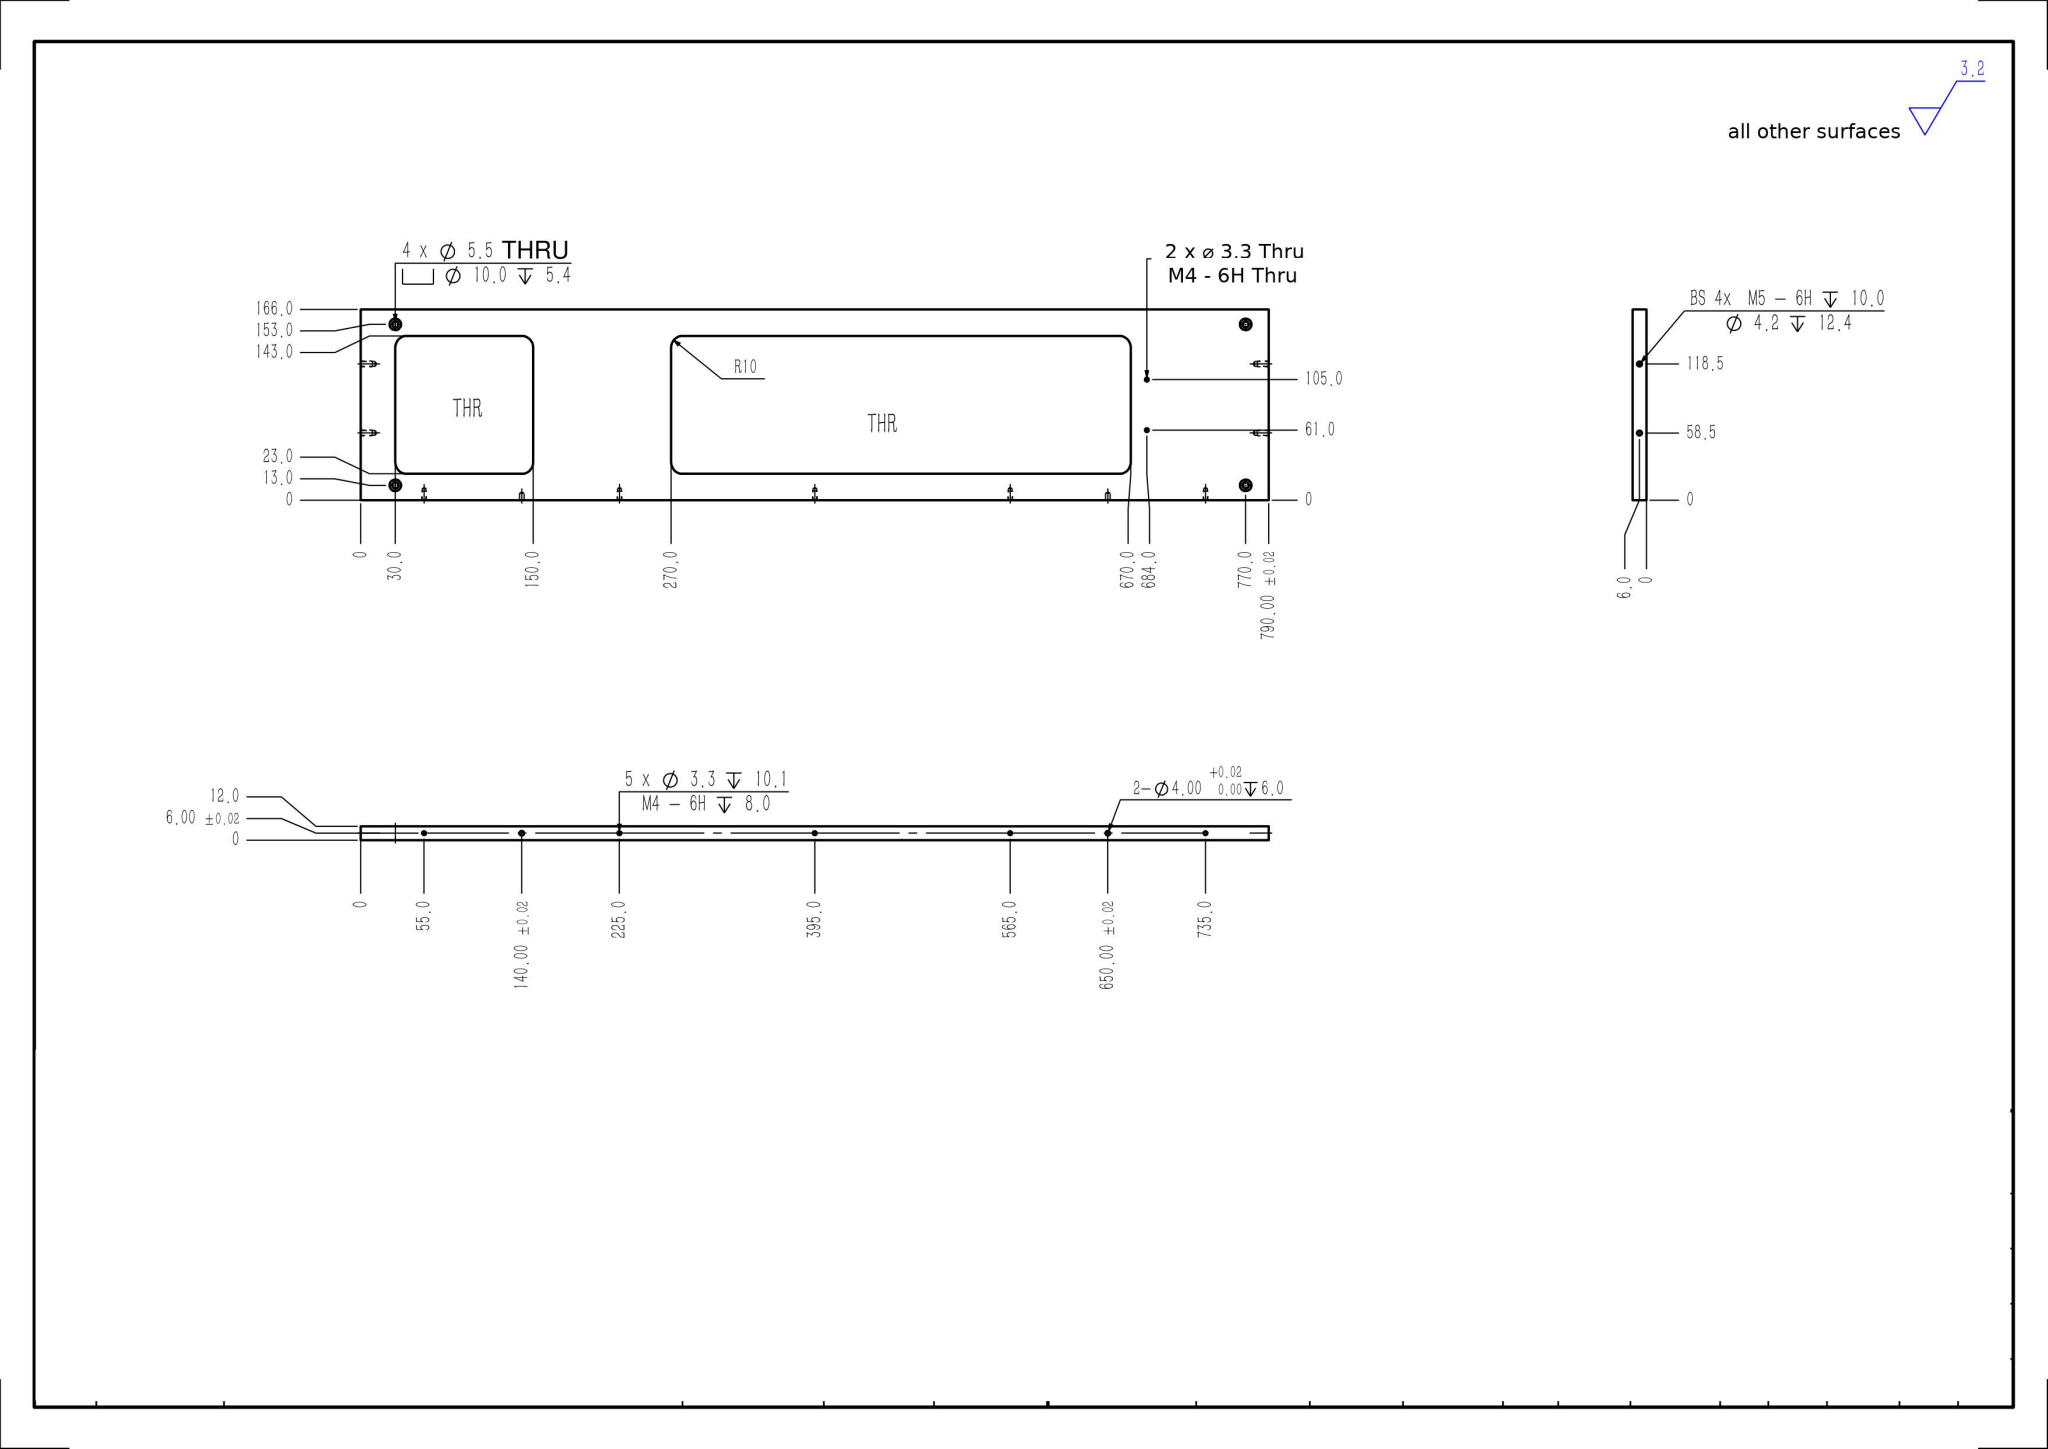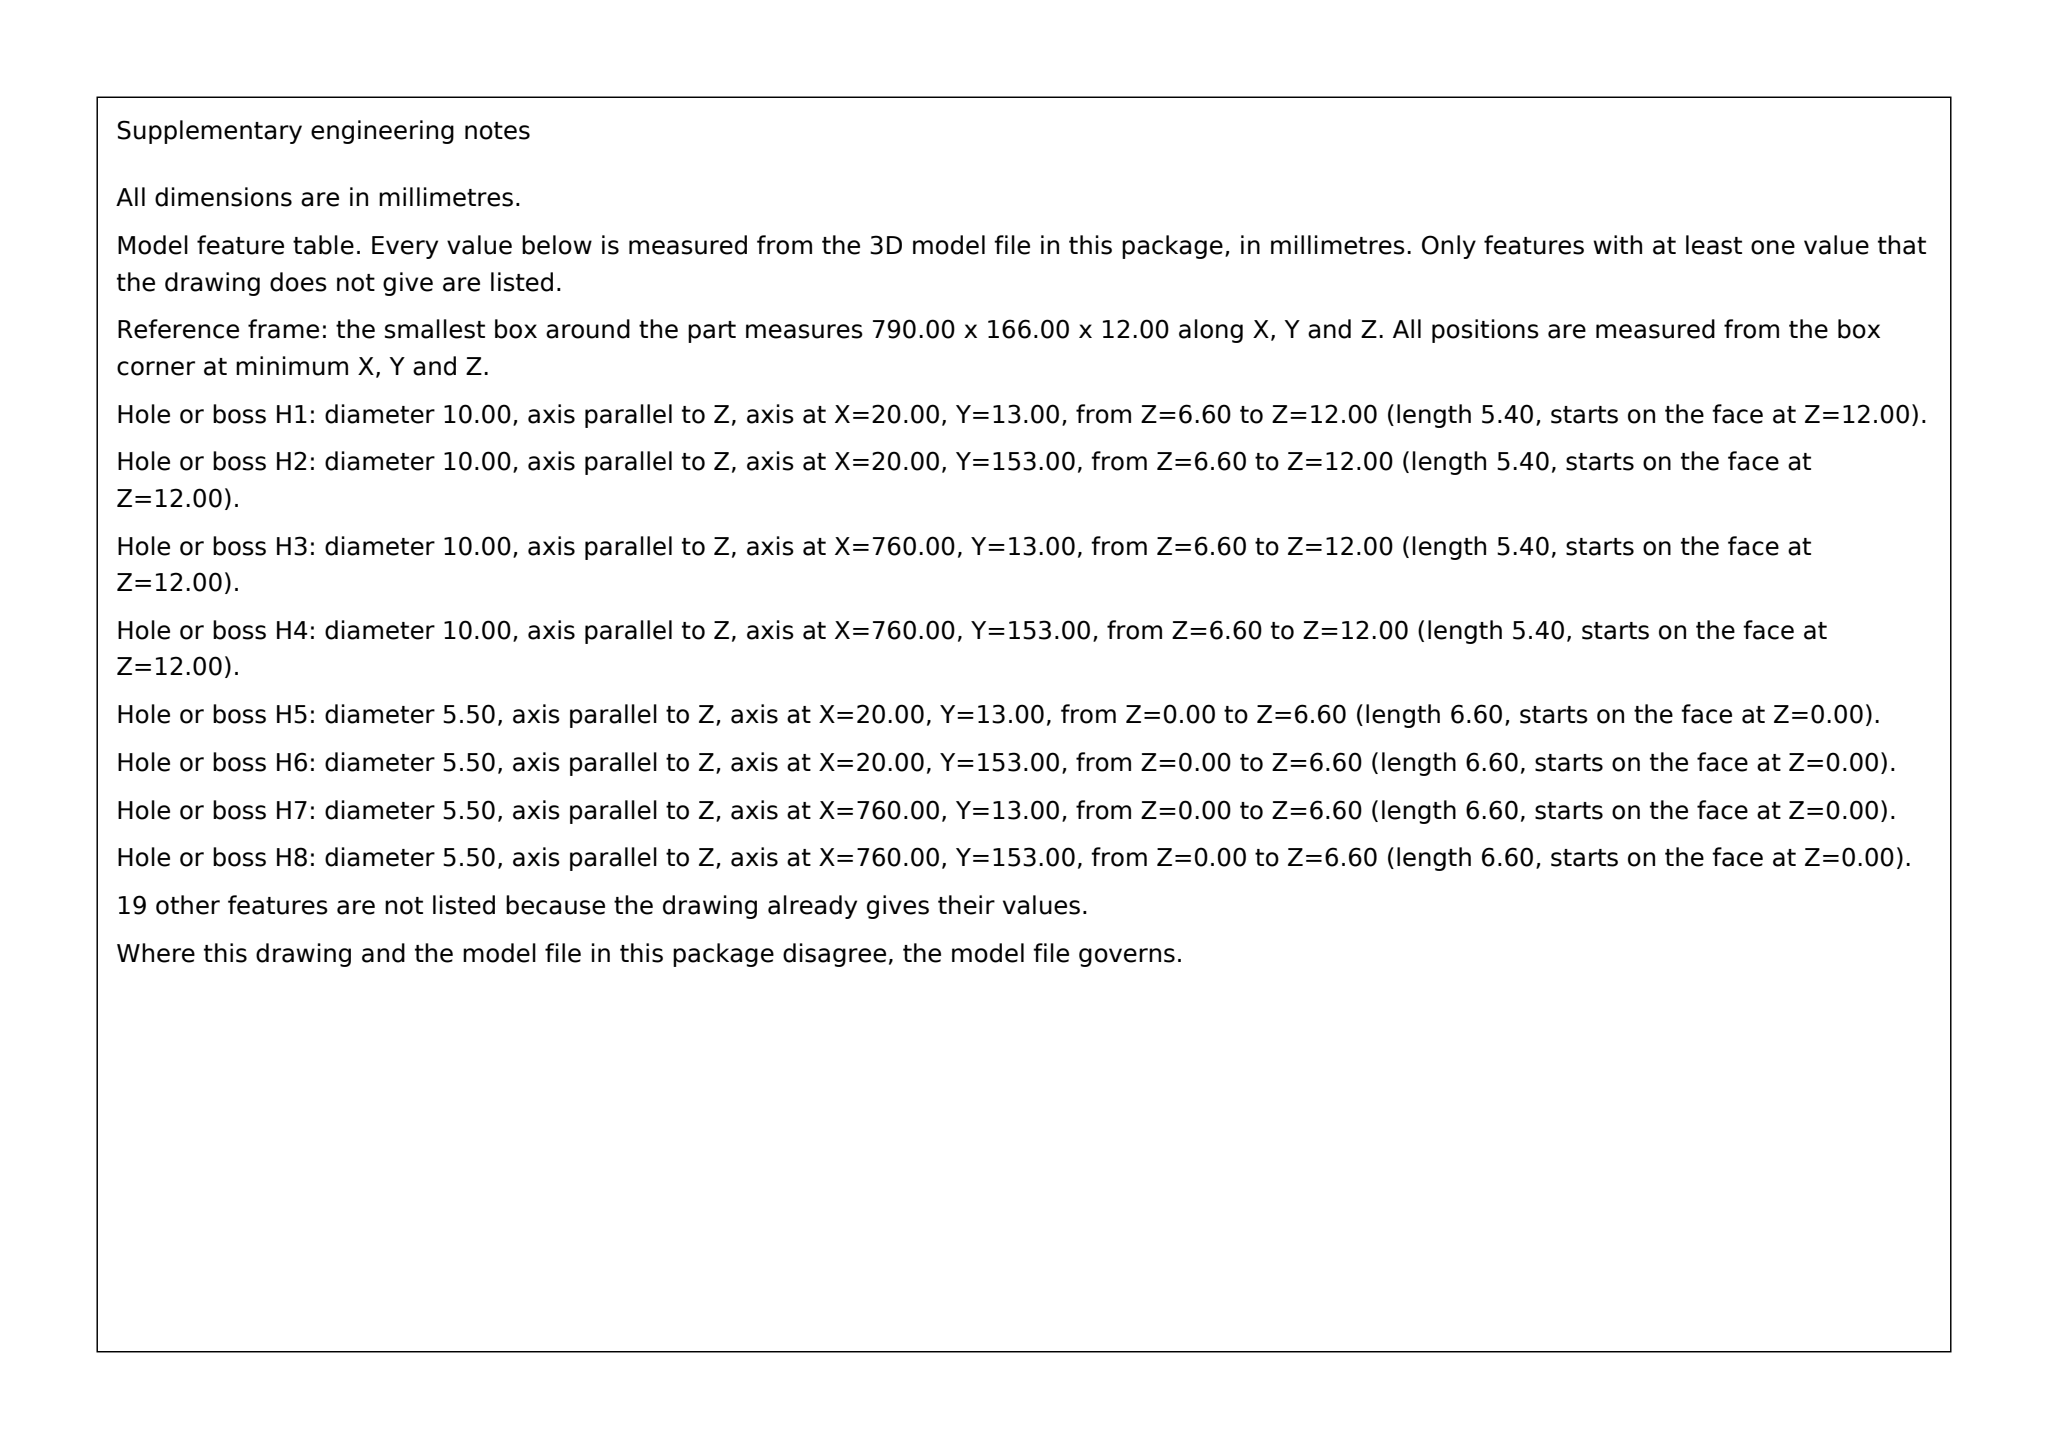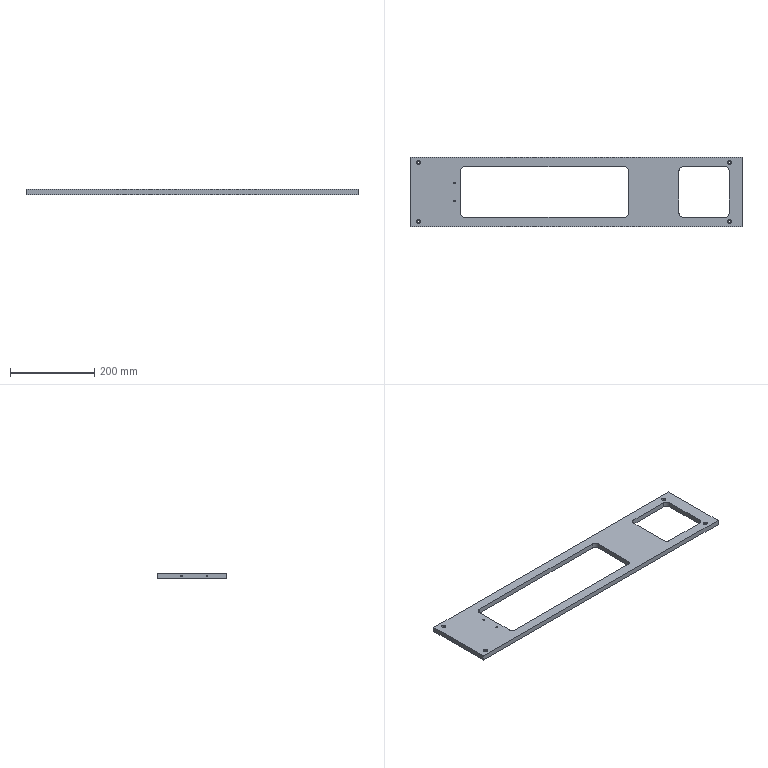Part | SolidWorks | mm | 1 solid | 90 faces | box 790 x 166 x 12 mm | volume 823094 mm3 | cylinder 50 | cone 22 | plane 18 | commonest cylinder face diameters 3.3 x14 4.2 x8 10 x8 5.5 x8 20 x8 4 x4
build123d program:
from build123d import *

# Parameters (mm, degrees)
SKETCH1_W                                       = 790
SKETCH1_H                                       = 166
BOSS_EXTRUDE1_DEPTH                             = 6
SKETCH63_W                                      = 120
SKETCH63_H                                      = 120
SKETCH63_W_2                                    = 400
CUT_EXTRUDE16_DEPTH                             = 404.804
FILLET6_R                                       = 10
M5_HEX_SOCKET_HEAD_CAP_SCREW_CBORE1_D           = 5.5
M5_HEX_SOCKET_HEAD_CAP_SCREW_CBORE1_CBORE_D     = 10
M5_HEX_SOCKET_HEAD_CAP_SCREW_CBORE1_CBORE_DEPTH = 5.4
M5_TAPPED_HOLE1_D                               = 4.2
M5_TAPPED_HOLE1_DEPTH                           = 12.4
M5_TAPPED_HOLE1_TIP                             = 1.262
M5_TAPPED_HOLE2_D                               = 4.2
M5_TAPPED_HOLE2_DEPTH                           = 12.4
M5_TAPPED_HOLE2_TIP                             = 1.262
M4_TAPPED_HOLE1_D                               = 3.3
M4_TAPPED_HOLE2_D                               = 3.3
M4_TAPPED_HOLE2_DEPTH                           = 10.1
M4_TAPPED_HOLE2_TIP                             = 0.9914
SIZE_MM_DOWEL_PIN_HOLE1_D                       = 4
SIZE_MM_DOWEL_PIN_HOLE1_DEPTH                   = 6
SIZE_MM_DOWEL_PIN_HOLE1_TIP                     = 1.202


with BuildPart() as part:
    # Sketch1 → Boss-Extrude1 (new, symmetric)
    with BuildSketch(Plane.XY):
        Rectangle(SKETCH1_W, SKETCH1_H)
    extrude(amount=BOSS_EXTRUDE1_DEPTH, both=True)

    # Sketch63 → Cut-Extrude16 (cut, through all)
    with BuildSketch(Plane(origin=(0, 0, -6), x_dir=(-1, 0, 0), z_dir=(0, 0, -1))):
        with Locations((-305, 0)):
            Rectangle(SKETCH63_W, SKETCH63_H)
        with Locations((75, 0)):
            Rectangle(SKETCH63_W_2, SKETCH63_H)
    extrude(amount=-CUT_EXTRUDE16_DEPTH, mode=Mode.SUBTRACT)

    # Fillet6
    fillet6_edges = [part.edges().sort_by_distance(p)[0] for p in [
        (245, 60, 0),
        (245, -60, 0),
        (365, -60, 0),
        (365, 60, 0),
        (-275, 60, 0),
        (-275, -60, 0),
        (125, -60, 0),
        (125, 60, 0),
    ]]
    fillet(fillet6_edges, radius=FILLET6_R)

    # M5 Hex Socket Head Cap Screw CBORE1 (through all)
    with Locations(Plane(origin=(0, 0, 6), x_dir=(-1, 0, 0), z_dir=(0, 0, 1))):
        with Locations((-365, -70), (-365, 70), (375, 70), (375, -70)):
            CounterBoreHole(M5_HEX_SOCKET_HEAD_CAP_SCREW_CBORE1_D / 2, M5_HEX_SOCKET_HEAD_CAP_SCREW_CBORE1_CBORE_D / 2, M5_HEX_SOCKET_HEAD_CAP_SCREW_CBORE1_CBORE_DEPTH)

    # M5 Tapped Hole1
    with Locations(Plane.ZY.offset(395)):
        with Locations((0, -35.5), (0, 24.5)):
            Hole(M5_TAPPED_HOLE1_D / 2, depth=M5_TAPPED_HOLE1_DEPTH)
            with Locations((0, 0, -(M5_TAPPED_HOLE1_DEPTH + M5_TAPPED_HOLE1_TIP / 2))):  # 118° drill point
                Cone(0, M5_TAPPED_HOLE1_D / 2, M5_TAPPED_HOLE1_TIP, mode=Mode.SUBTRACT)

    # M5 Tapped Hole2
    with Locations(Plane(origin=(395, 0, 0), x_dir=(0, 0, -1), z_dir=(1, 0, 0))):
        with Locations((0, 24.5), (0, -35.5)):
            Hole(M5_TAPPED_HOLE2_D / 2, depth=M5_TAPPED_HOLE2_DEPTH)
            with Locations((0, 0, -(M5_TAPPED_HOLE2_DEPTH + M5_TAPPED_HOLE2_TIP / 2))):  # 118° drill point
                Cone(0, M5_TAPPED_HOLE2_D / 2, M5_TAPPED_HOLE2_TIP, mode=Mode.SUBTRACT)

    # M4 Tapped Hole1 (through all)
    with Locations(Plane(origin=(0, 0, -6), x_dir=(-1, 0, 0), z_dir=(0, 0, -1))):
        with Locations((289, 22), (289, -22)):
            Hole(M4_TAPPED_HOLE1_D / 2)

    # M4 Tapped Hole2
    with Locations(Plane(origin=(0, 83, 0), x_dir=(1, 0, 0), z_dir=(0, 1, 0))):
        with Locations((-340, 0), (-170, 0), (0, 0), (170, 0), (340, 0)):
            Hole(M4_TAPPED_HOLE2_D / 2, depth=M4_TAPPED_HOLE2_DEPTH)
            with Locations((0, 0, -(M4_TAPPED_HOLE2_DEPTH + M4_TAPPED_HOLE2_TIP / 2))):  # 118° drill point
                Cone(0, M4_TAPPED_HOLE2_D / 2, M4_TAPPED_HOLE2_TIP, mode=Mode.SUBTRACT)

    # Size mm Dowel Pin Hole1
    with Locations(Plane(origin=(0, 83, 0), x_dir=(1, 0, 0), z_dir=(0, 1, 0))):
        with Locations((-255, 0), (255, 0)):
            Hole(SIZE_MM_DOWEL_PIN_HOLE1_D / 2, depth=SIZE_MM_DOWEL_PIN_HOLE1_DEPTH)
            with Locations((0, 0, -(SIZE_MM_DOWEL_PIN_HOLE1_DEPTH + SIZE_MM_DOWEL_PIN_HOLE1_TIP / 2))):  # 118° drill point
                Cone(0, SIZE_MM_DOWEL_PIN_HOLE1_D / 2, SIZE_MM_DOWEL_PIN_HOLE1_TIP, mode=Mode.SUBTRACT)


solid = part.part